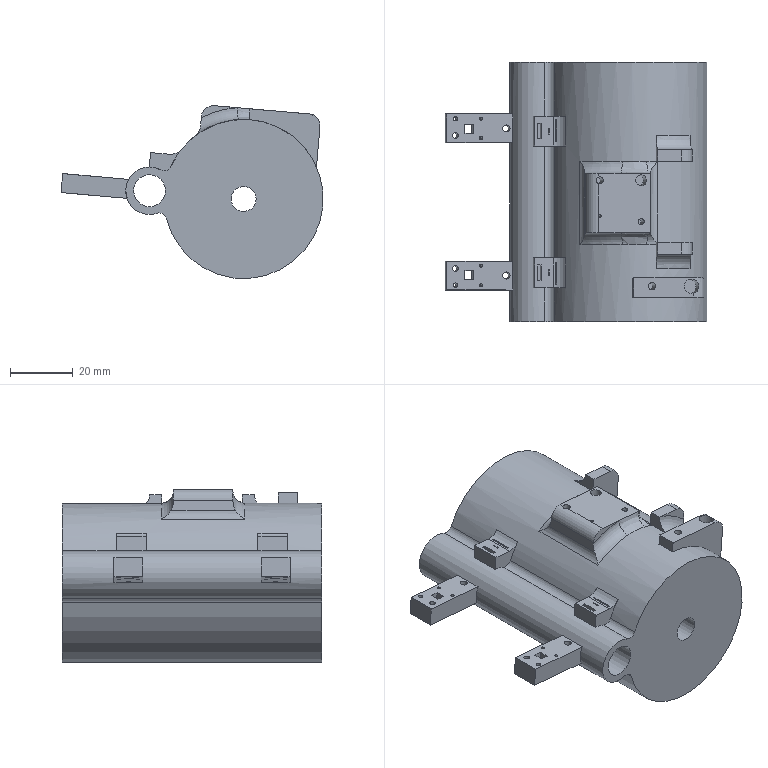Component | NX | LUN_GU | 1 solid | 126 faces | volume 176927 mm3 | plane 86 | cylinder 32 | torus 6 | spline 2 | commonest cylinder face diameters 7.6 x6 4.56 x4 2.291 x3 1.018 x2 1.803 x2 1.374 x2 0.945 x2 9.12 x2